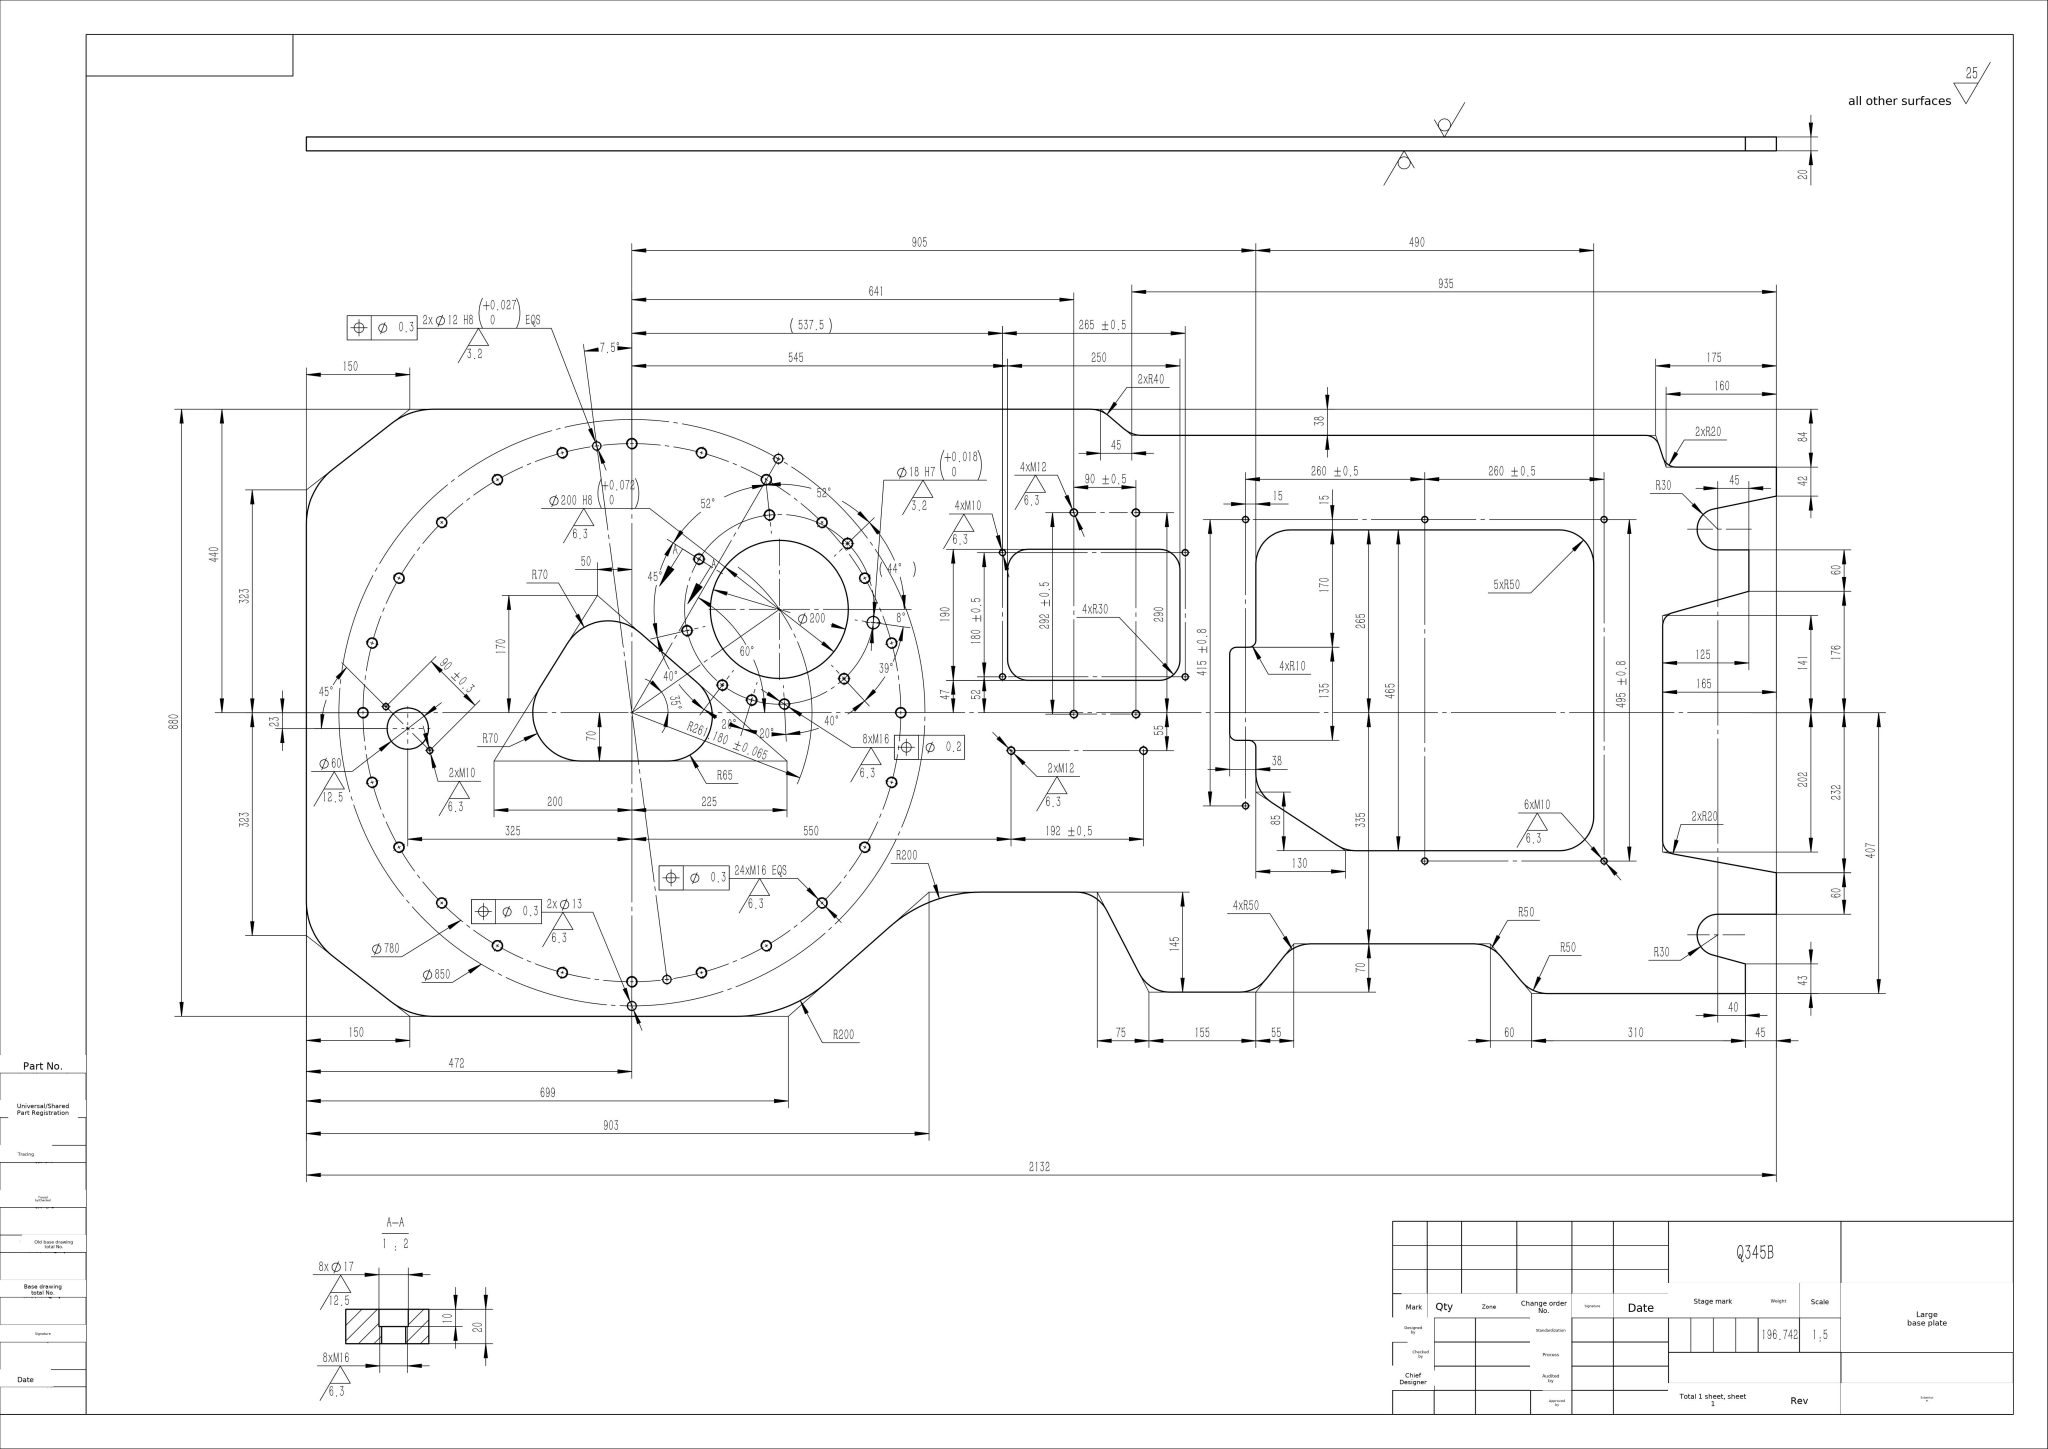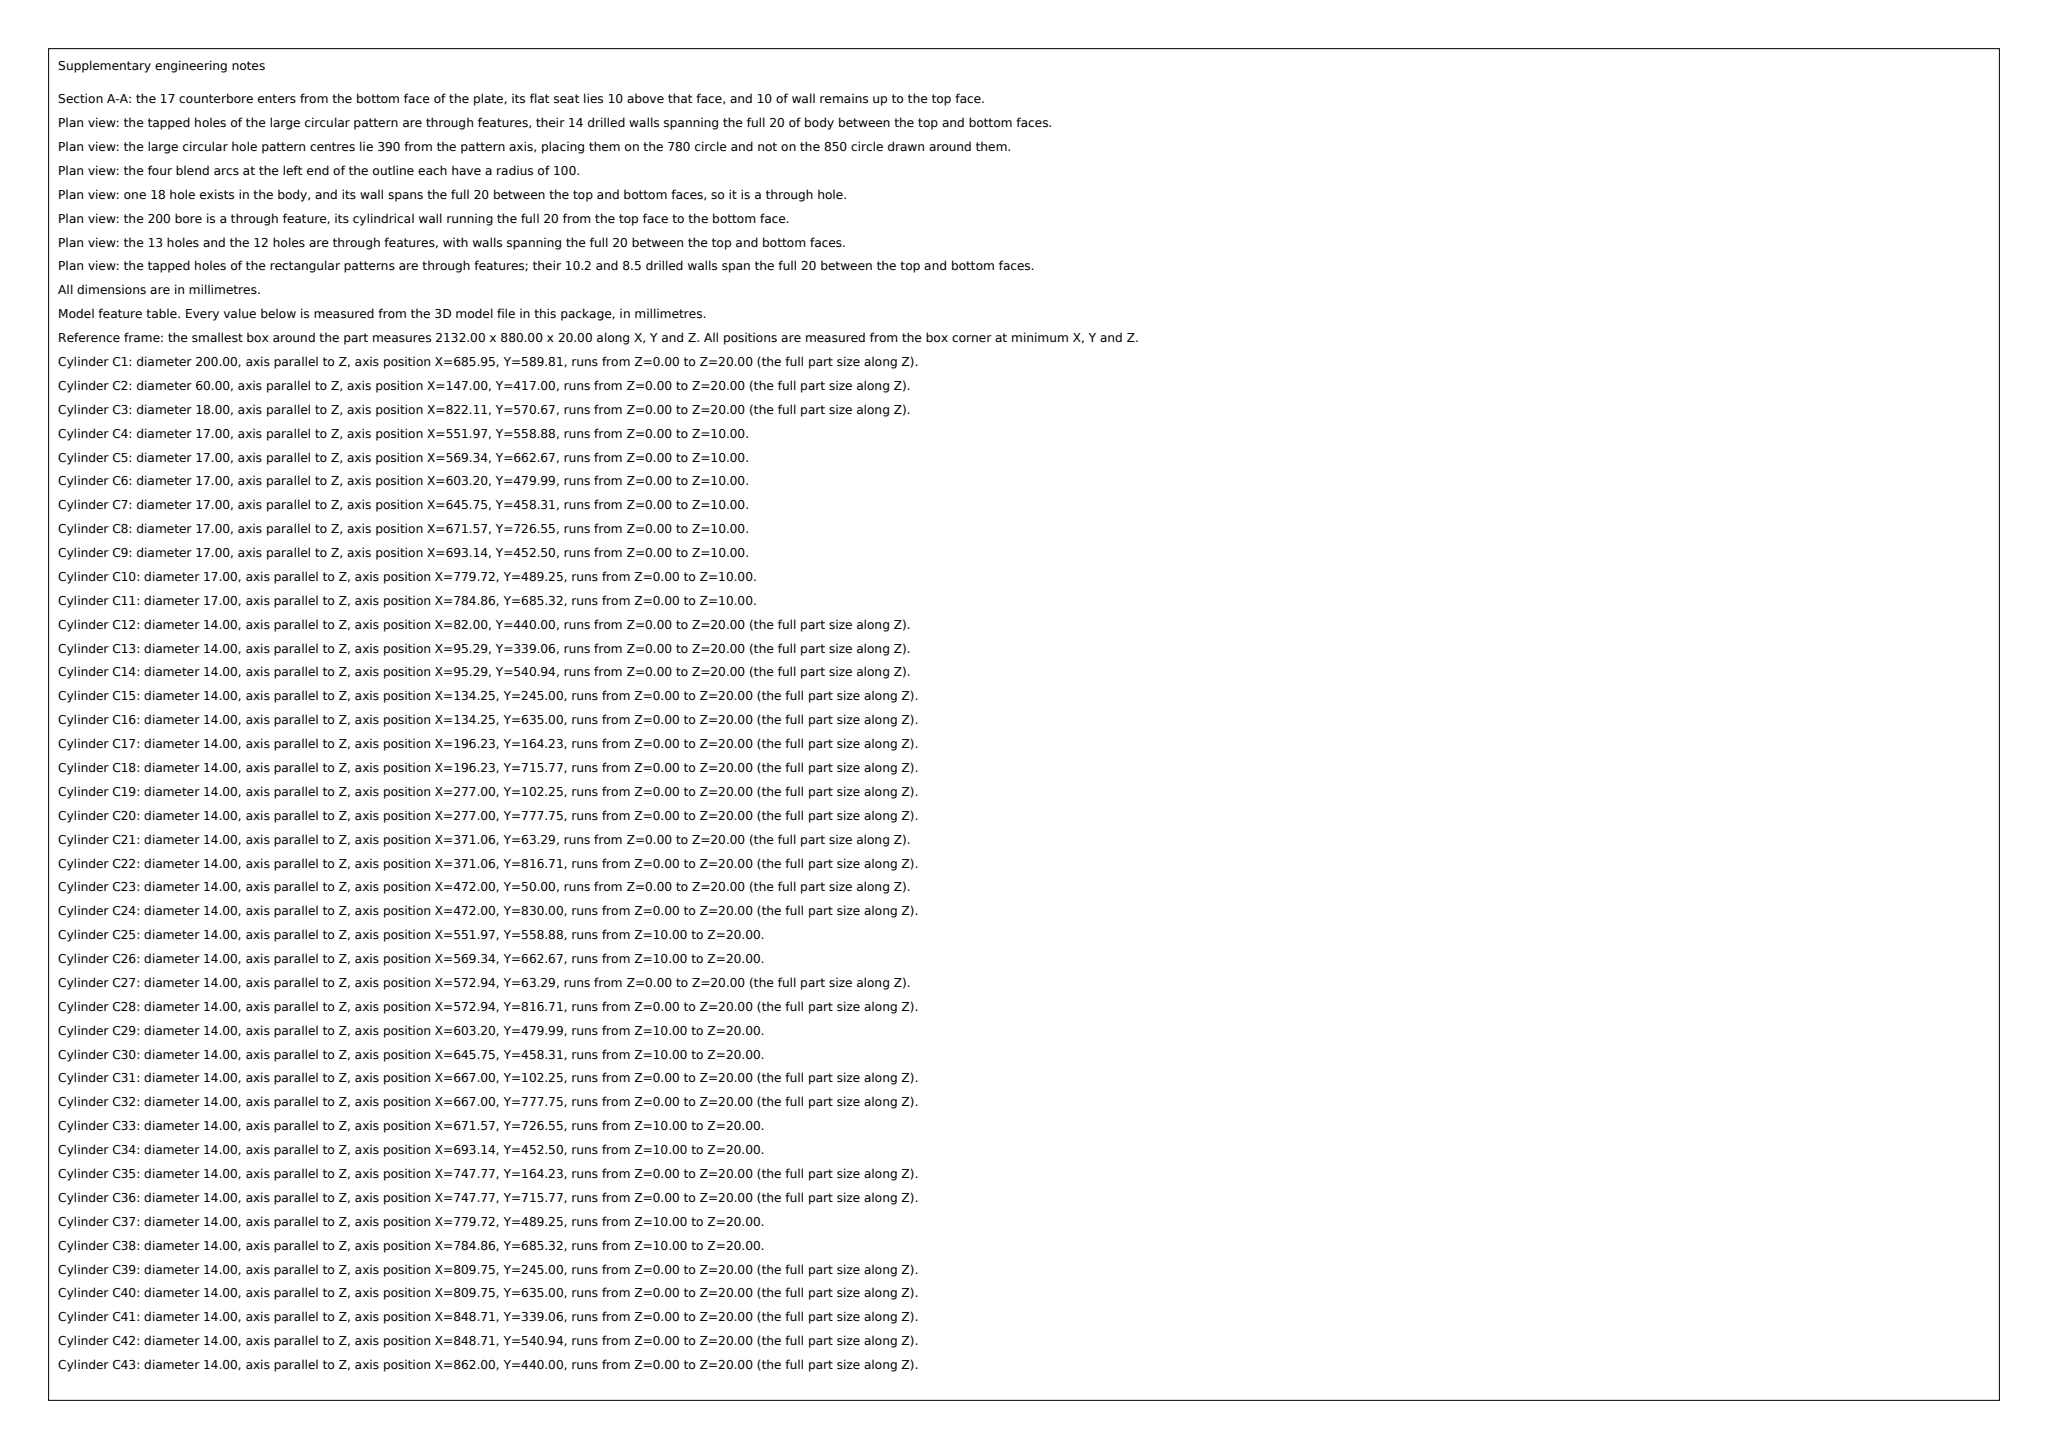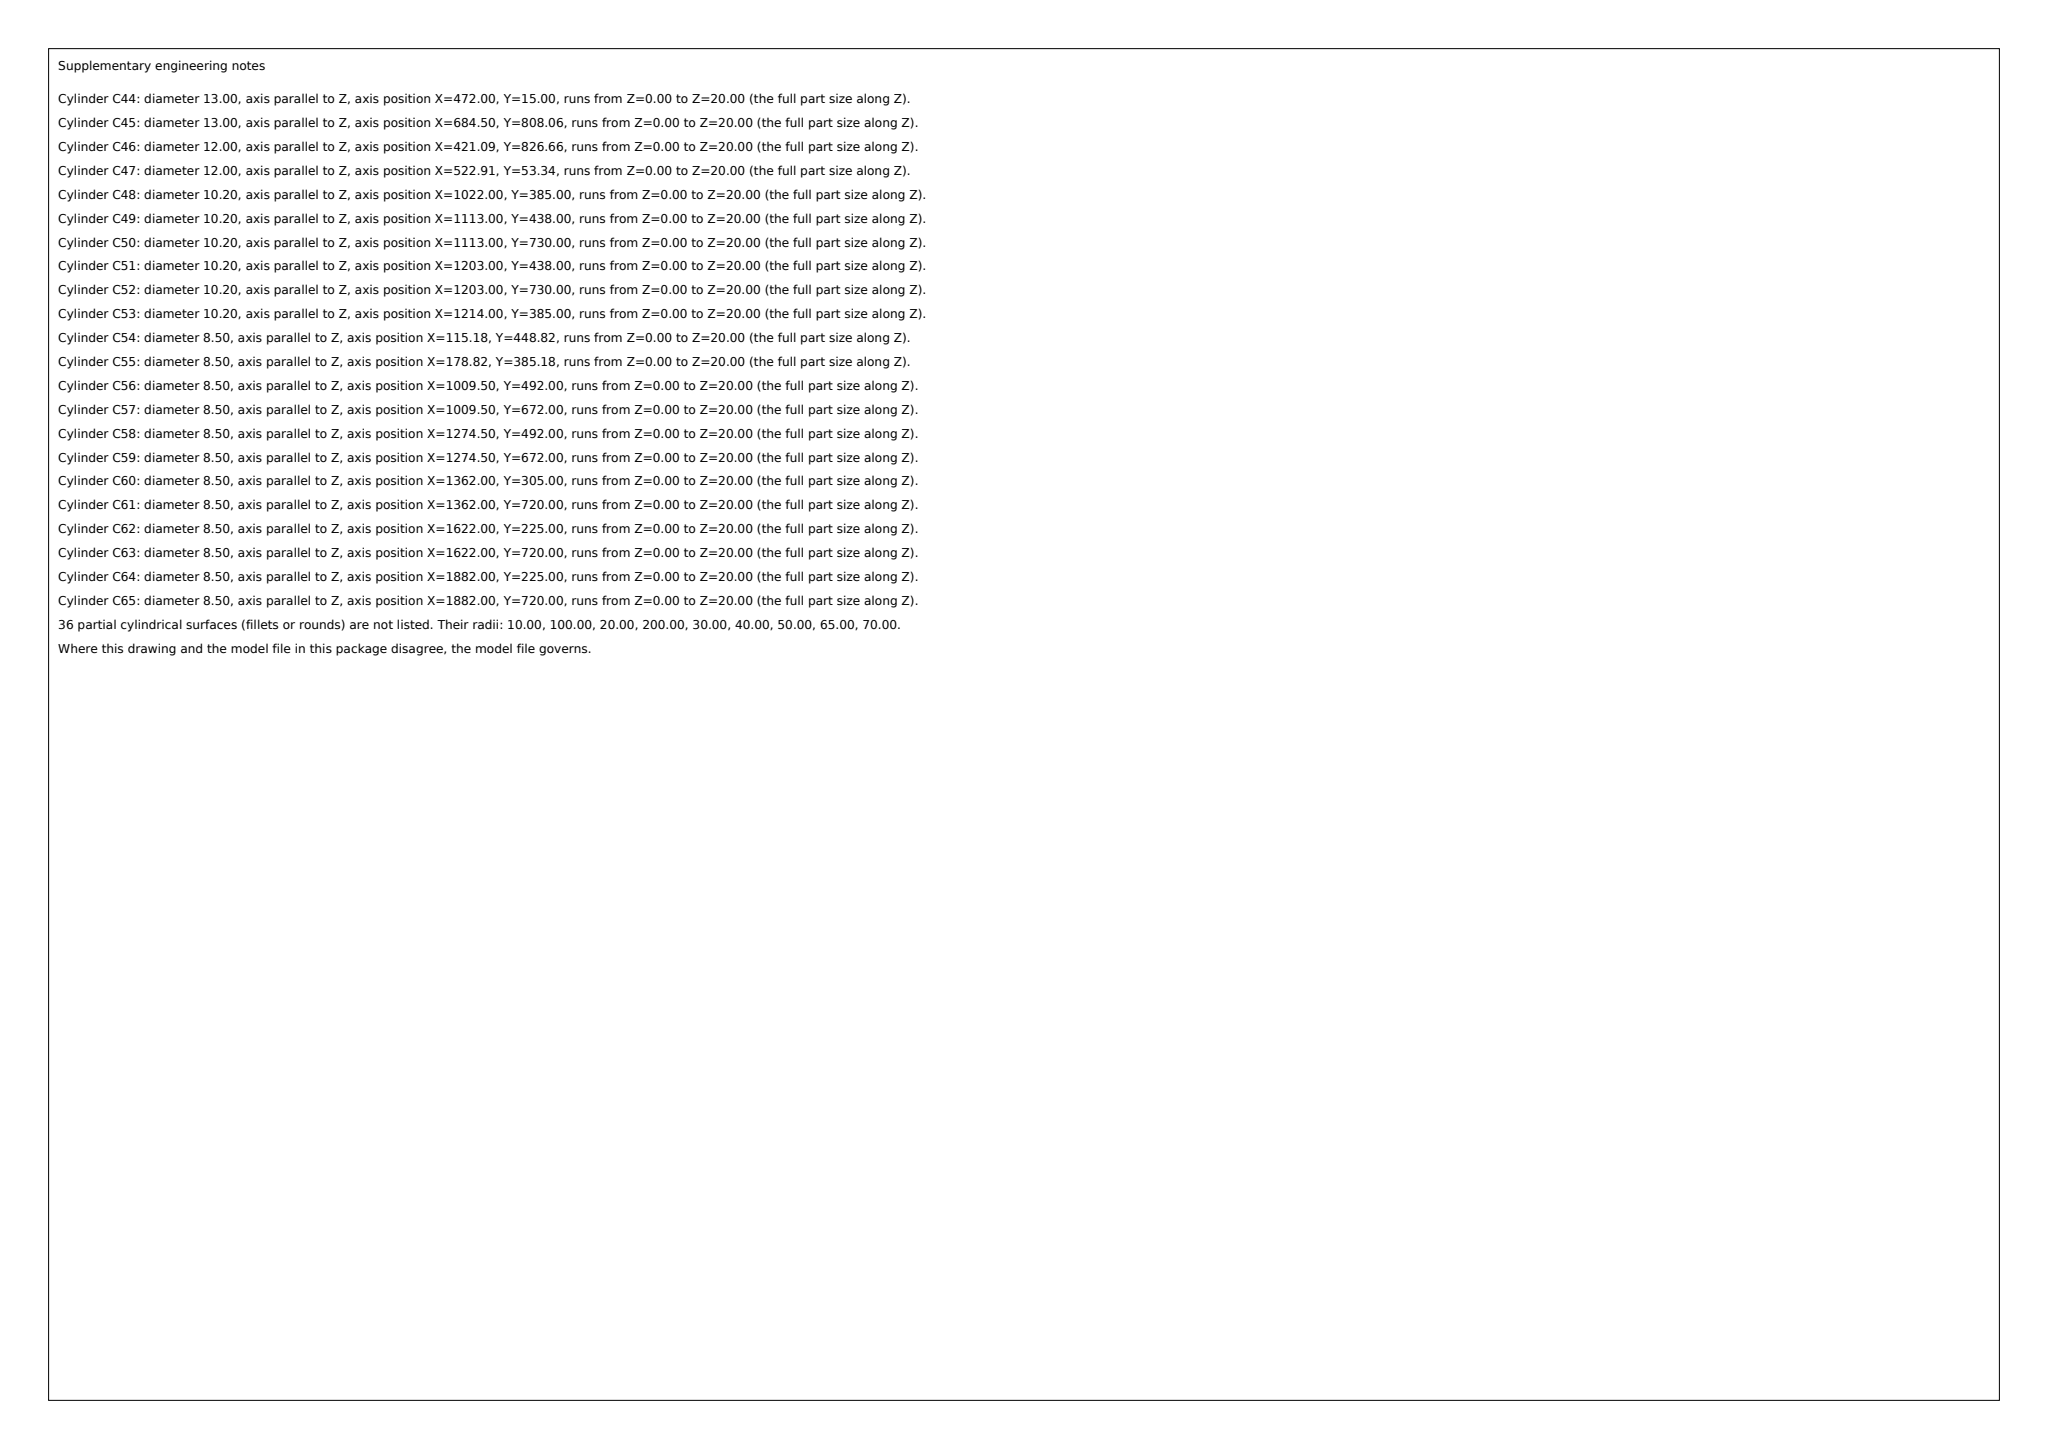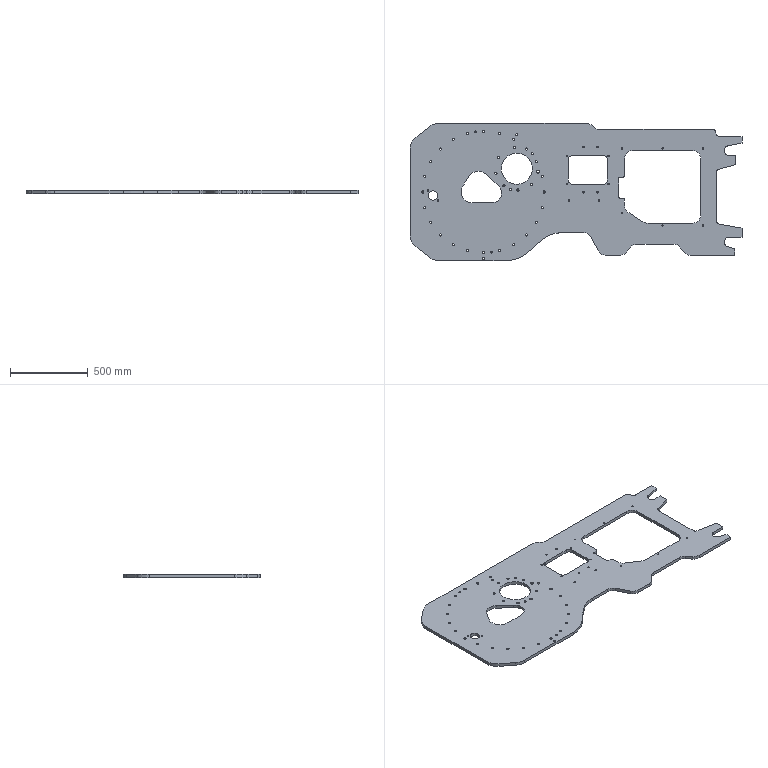Part | SolidWorks | mm | material Q345B | 1 solid | 223 faces | box 2132 x 880 x 20 mm | volume 25062640 mm3 | cylinder 169 | plane 54 | commonest cylinder face diameters 14 x64 8.5 x24 17 x16 10.2 x12 100 x11 60 x10 200 x6 12 x4
build123d program:
from build123d import *

# Parameters (mm, degrees)
SKETCH1_R           = 100
BOSS_EXTRUDE1_DEPTH = 20
SKETCH2_R           = 30
SKETCH2_R_2         = 9
SKETCH2_R_3         = 6
SKETCH2_R_4         = 6.5
CUT_EXTRUDE1_DEPTH  = 20
M16_TAPPED_HOLE1_D  = 14
CIRPATTERN1_COUNT   = 24
M10_TAPPED_HOLE1_D  = 8.5
M16_TAPPED_HOLE2_D  = 14
M10_TAPPED_HOLE2_D  = 8.5
M12_TAPPED_HOLE1_D  = 10.2
M10_TAPPED_HOLE3_D  = 8.5
SKETCH11_R          = 8.5
CUT_EXTRUDE2_DEPTH  = 10


with BuildPart() as part:
    # Sketch1 → Boss-Extrude1 (new body)
    with BuildSketch(Plane.XY):
        with BuildLine():
            Line((-472, 274.177), (-472, -274.177))
            ThreePointArc((-472, -274.177), (-461.862, -318.05), (-433.503, -353.028))
            Line((-433.503, -353.028), (-349.115, -418.85))
            ThreePointArc((-349.115, -418.85), (-320.131, -434.565), (-287.612, -440))
            Line((-287.612, -440), (151.379, -440))
            ThreePointArc((151.379, -440), (222.113, -427.074), (283.703, -389.968))
            Line((283.703, -389.968), (374.297, -310.032))
            ThreePointArc((374.297, -310.032), (435.887, -272.926), (506.621, -260))
            Line((506.621, -260), (644.57, -260))
            ThreePointArc((644.57, -260), (670.564, -267.288), (688.98, -287.029))
            Line((688.98, -287.029), (736.02, -377.971))
            ThreePointArc((736.02, -377.971), (754.436, -397.712), (780.43, -405))
            Line((780.43, -405), (880.698, -405))
            ThreePointArc((880.698, -405), (902.555, -399.97), (920.014, -385.891))
            Line((920.014, -385.891), (944.986, -354.109))
            ThreePointArc((944.986, -354.109), (962.445, -340.03), (984.302, -335))
            Line((984.302, -335), (1221.581, -335))
            ThreePointArc((1221.581, -335), (1242.789, -339.721), (1259.992, -352.991))
            Line((1259.992, -352.991), (1290.008, -389.009))
            ThreePointArc((1290.008, -389.009), (1307.211, -402.279), (1328.419, -407))
            Line((1328.419, -407), (1615, -407))
            Line((1615, -407), (1615, -364))
            Line((1615, -364), (1567.109, -350.944))
            ThreePointArc((1567.109, -350.944), (1545.265, -318.019), (1575, -292))
            Line((1575, -292), (1660, -292))
            Line((1660, -292), (1660, -232))
            Line((1660, -232), (1511.422, -204.986))
            ThreePointArc((1511.422, -204.986), (1499.645, -198.123), (1495, -185.308))
            Line((1495, -185.308), (1495, 125.831))
            ThreePointArc((1495, 125.831), (1499.065, 137.917), (1509.607, 145.09))
            Line((1509.607, 145.09), (1620, 176))
            Line((1620, 176), (1620, 236))
            Line((1620, 236), (1575, 236))
            ThreePointArc((1575, 236), (1545.152, 262.98), (1568.99, 295.392))
            Line((1568.99, 295.392), (1660, 314))
            Line((1660, 314), (1660, 356))
            Line((1660, 356), (1514.515, 356))
            ThreePointArc((1514.515, 356), (1502.768, 359.813), (1495.5, 369.8))
            Line((1495.5, 369.8), (1489.5, 388.2))
            ThreePointArc((1489.5, 388.2), (1482.232, 398.187), (1470.485, 402))
            Line((1470.485, 402), (739.63, 402))
            ThreePointArc((739.63, 402), (725.89, 404.434), (713.822, 411.439))
            Line((713.822, 411.439), (691.178, 430.561))
            ThreePointArc((691.178, 430.561), (679.11, 437.566), (665.37, 440))
            Line((665.37, 440), (-287.612, 440))
            ThreePointArc((-287.612, 440), (-320.131, 434.565), (-349.115, 418.85))
            Line((-349.115, 418.85), (-433.503, 353.028))
            ThreePointArc((-433.503, 353.028), (-461.862, 318.05), (-472, 274.177))
        make_face()
        with Locations((213.946, 149.807)):
            Circle(SKETCH1_R, mode=Mode.SUBTRACT)
        with BuildLine():
            Line((-93.52, 100.367), (-133.063, 37.1))
            ThreePointArc((-133.063, 37.1), (-134.928, -33.934), (-73.703, -70))
            Line((-73.703, -70), (51.667, -70))
            ThreePointArc((51.667, -70), (112.528, -27.823), (94.406, 43.973))
            Line((94.406, 43.973), (11.867, 116.007))
            ThreePointArc((11.867, 116.007), (-44.436, 132.509), (-93.52, 100.367))
        make_face(mode=Mode.SUBTRACT)
        with BuildLine():
            Line((575, 237), (765, 237))
            ThreePointArc((765, 237), (786.213, 228.213), (795, 207))
            Line((795, 207), (795, 77))
            ThreePointArc((795, 77), (786.213, 55.787), (765, 47))
            Line((765, 47), (575, 47))
            ThreePointArc((575, 47), (553.787, 55.787), (545, 77))
            Line((545, 77), (545, 207))
            ThreePointArc((545, 207), (553.787, 228.213), (575, 237))
        make_face(mode=Mode.SUBTRACT)
        with BuildLine():
            Line((877, 95), (895, 95))
            ThreePointArc((895, 95), (902.071, 97.929), (905, 105))
            Line((905, 105), (905, 215))
            ThreePointArc((905, 215), (919.645, 250.355), (955, 265))
            Line((955, 265), (1345, 265))
            ThreePointArc((1345, 265), (1380.355, 250.355), (1395, 215))
            Line((1395, 215), (1395, -150))
            ThreePointArc((1395, -150), (1380.355, -185.355), (1345, -200))
            Line((1345, -200), (1049.895, -200))
            ThreePointArc((1049.895, -200), (1035.62, -197.919), (1022.533, -191.848))
            Line((1022.533, -191.848), (927.638, -129.801))
            ThreePointArc((927.638, -129.801), (911.022, -111.742), (905, -87.953))
            Line((905, -87.953), (905, -50))
            ThreePointArc((905, -50), (902.071, -42.929), (895, -40))
            Line((895, -40), (877, -40))
            ThreePointArc((877, -40), (869.929, -37.071), (867, -30))
            Line((867, -30), (867, 85))
            ThreePointArc((867, 85), (869.929, 92.071), (877, 95))
        make_face(mode=Mode.SUBTRACT)
    extrude(amount=BOSS_EXTRUDE1_DEPTH)

    # Sketch2 → Cut-Extrude1 (cut)
    with BuildSketch(Plane.XY.offset(20)):
        with Locations((-325, -23)):
            Circle(SKETCH2_R)
        with Locations((350.108, 130.67)):
            Circle(SKETCH2_R_2)
        with Locations((-50.905, 386.663)):
            Circle(SKETCH2_R_3)
        with Locations((50.905, -386.663)):
            Circle(SKETCH2_R_3)
        with Locations((0, -425)):
            Circle(SKETCH2_R_4)
        with Locations((212.5, 368.061)):
            Circle(SKETCH2_R_4)
    extrude(amount=-CUT_EXTRUDE1_DEPTH, mode=Mode.SUBTRACT)

    # M16 Tapped Hole1 (through all)
    with Locations(Plane(origin=(-390, 0, 20), x_dir=(1, 0, 0), z_dir=(0, 0, 1))):
        with Locations((0, 0)):
            m16_tapped_hole1 = Hole(M16_TAPPED_HOLE1_D / 2)

    # CirPattern1: M16 Tapped Hole1 ×24 about axis
    cirpattern1_axis = Axis((0, 0, 0), (0, 0, 1))
    for i in range(1, CIRPATTERN1_COUNT):
        add(m16_tapped_hole1.rotate(cirpattern1_axis, i * 360 / CIRPATTERN1_COUNT), mode=Mode.SUBTRACT)

    # M10 Tapped Hole1 (through all)
    with Locations(Plane(origin=(-356.82, 8.82, 20), x_dir=(1, 0, 0), z_dir=(0, 0, 1))):
        with Locations((0, 0), (63.64, -63.64)):
            Hole(M10_TAPPED_HOLE1_D / 2)

    # M16 Tapped Hole2 (through all)
    with Locations(Plane(origin=(97.34, 222.671, 20), x_dir=(1, 0, 0), z_dir=(0, 0, 1))):
        with Locations((0, 0), (102.234, 63.883), (215.516, 22.652), (210.381, -173.425), (123.803, -210.175), (76.406, -204.356), (33.857, -182.676), (-17.369, -103.795)):
            Hole(M16_TAPPED_HOLE2_D / 2)

    # M10 Tapped Hole2 (through all)
    with Locations(Plane(origin=(537.5, 232, 20), x_dir=(1, 0, 0), z_dir=(0, 0, 1))):
        with Locations((0, 0), (265, 0), (265, -180), (0, -180)):
            Hole(M10_TAPPED_HOLE2_D / 2)

    # M12 Tapped Hole1 (through all)
    with Locations(Plane(origin=(550, -55, 20), x_dir=(1, 0, 0), z_dir=(0, 0, 1))):
        with Locations((0, 0), (192, 0), (181, 53), (91, 53), (181, 345), (91, 345)):
            Hole(M12_TAPPED_HOLE1_D / 2)

    # M10 Tapped Hole3 (through all)
    with Locations(Plane(origin=(890, 280, 20), x_dir=(1, 0, 0), z_dir=(0, 0, 1))):
        with Locations((0, 0), (260, 0), (520, 0), (520, -495), (260, -495), (0, -415)):
            Hole(M10_TAPPED_HOLE3_D / 2)

    # Sketch11 → Cut-Extrude2 (cut)
    with BuildSketch(Plane(origin=(0, 0, 0), x_dir=(-1, 0, 0), z_dir=(0, 0, -1))):
        with Locations((-307.721, 49.246)):
            Circle(SKETCH11_R)
        with Locations((-221.142, 12.495)):
            Circle(SKETCH11_R)
        with Locations((-173.745, 18.315)):
            Circle(SKETCH11_R)
        with Locations((-131.197, 39.994)):
            Circle(SKETCH11_R)
        with Locations((-79.97, 118.876)):
            Circle(SKETCH11_R)
        with Locations((-97.34, 222.671)):
            Circle(SKETCH11_R)
        with Locations((-199.573, 286.553)):
            Circle(SKETCH11_R)
        with Locations((-312.855, 245.322)):
            Circle(SKETCH11_R)
    extrude(amount=-CUT_EXTRUDE2_DEPTH, mode=Mode.SUBTRACT)


solid = part.part